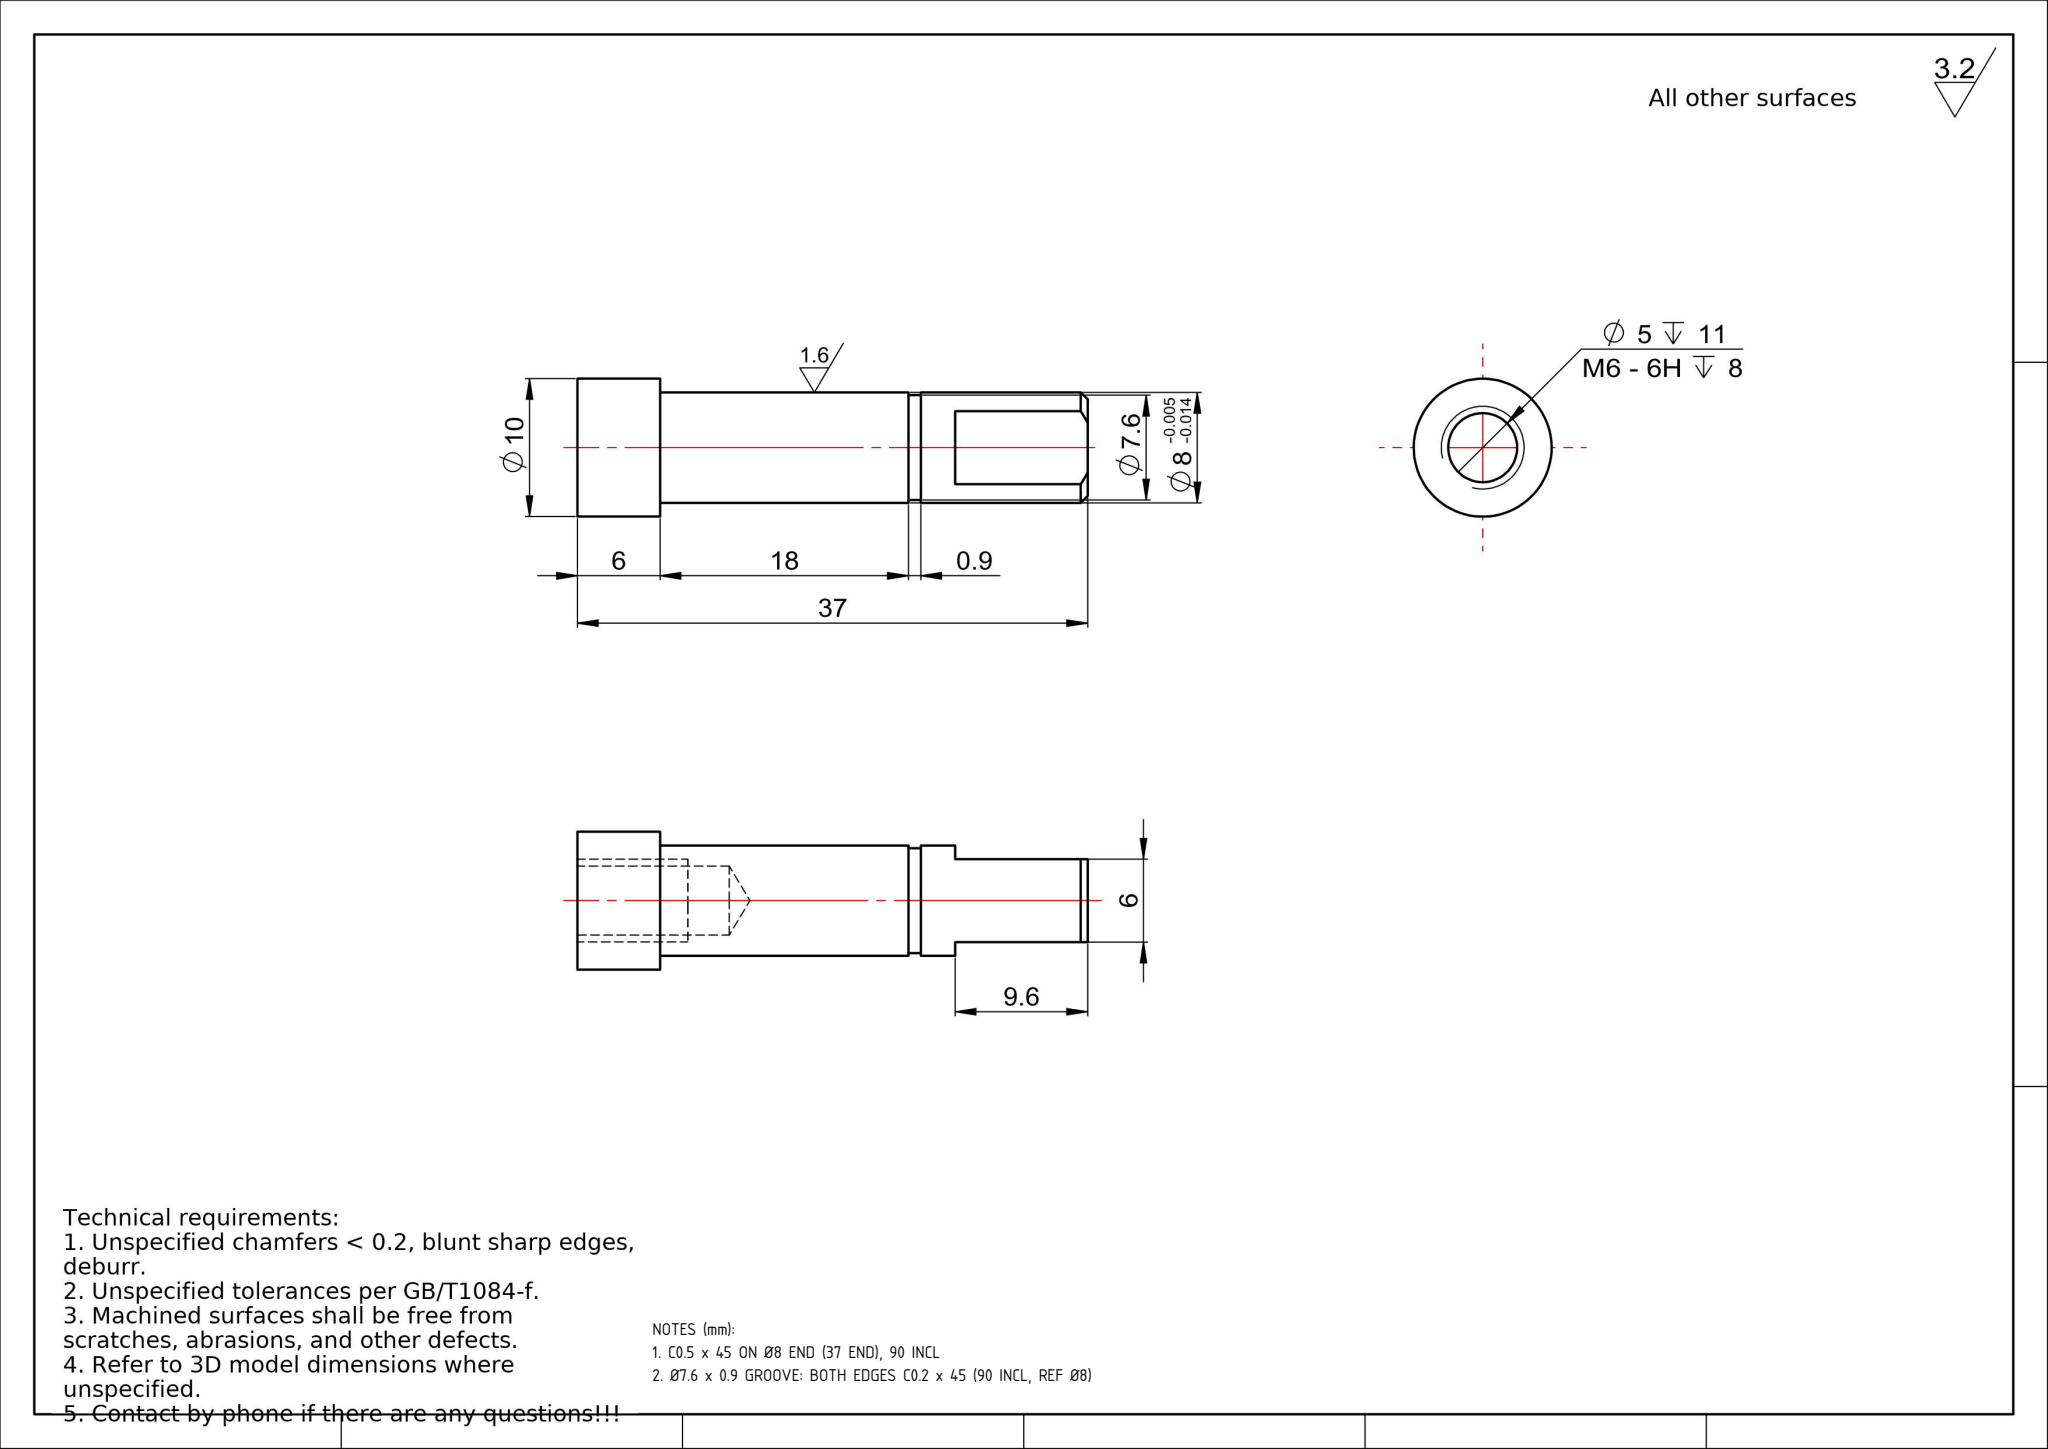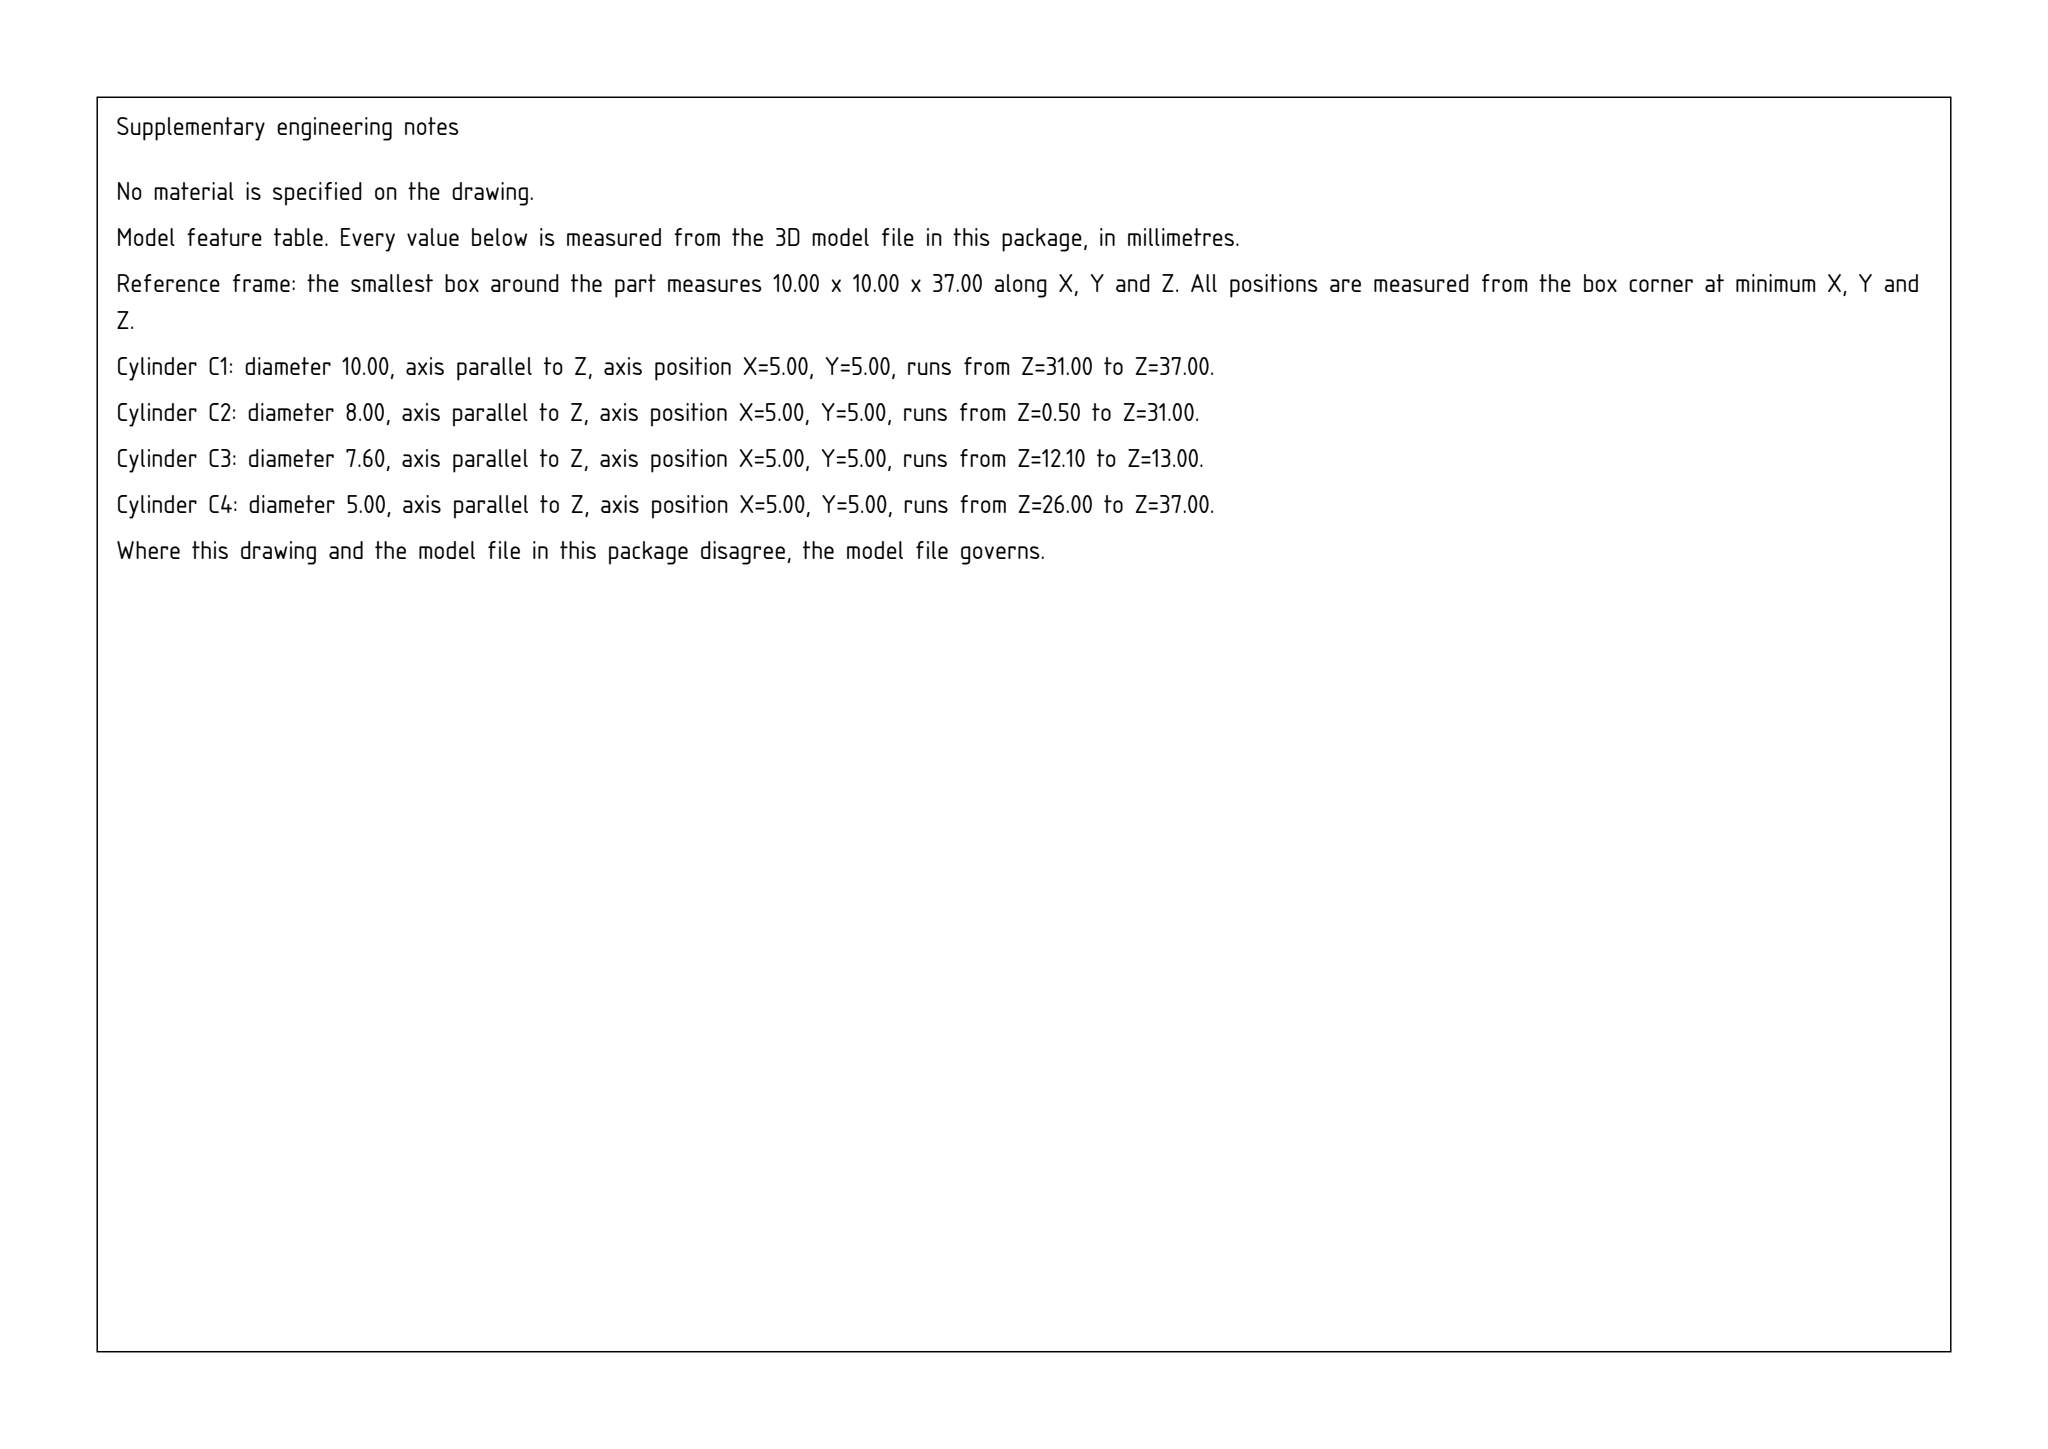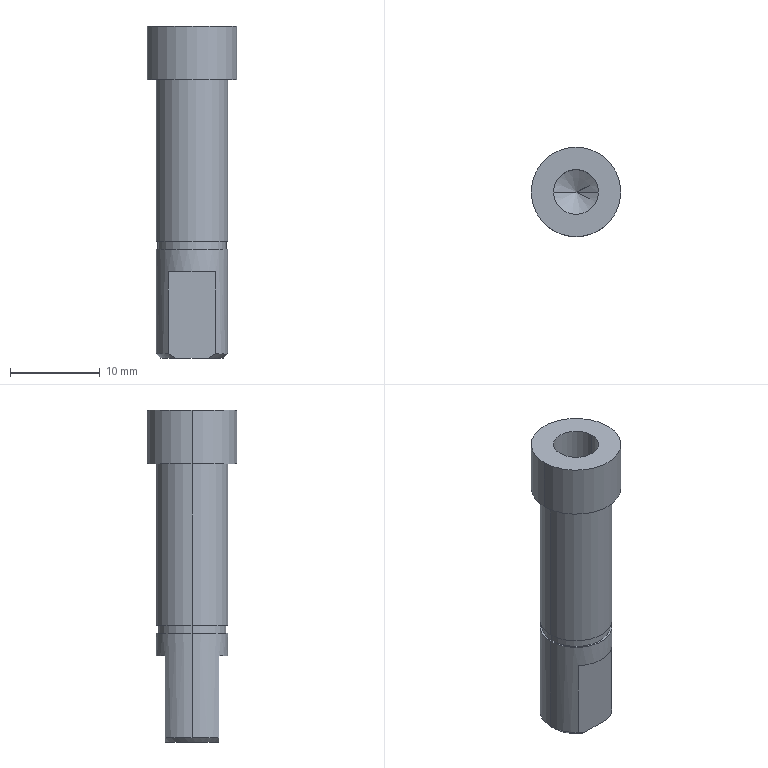Part | SolidWorks | mm | 1 solid | 24 faces | box 10 x 10 x 37 mm | volume 1728 mm3 | cylinder 10 | plane 9 | cone 5 | commonest cylinder face diameters 8 x4 5 x2 10 x2 7.6 x2
Drawing notes:
C0.5 x 45 ON Ø8 END (37 END), 90 INCL | from the solid: cones[included_angle,ref_dia]=90.0 @ ref dia 8.0 at z=37 end face of Ø8 shaft
Ø7.6 x 0.9 GROOVE: BOTH EDGES C0.2 x 45 (90 INCL, REF Ø8) | from the solid: cyl Ø7.6 L0.9 between z=12.1 and 13.0; 90 deg cones ref Ø8; (8-7.6)/2=0.2 radial
build123d program:
from build123d import *

# Parameters (mm, degrees)
SKETCH1_R               = 4
BOSS_EXTRUDE1_DEPTH     = 12.1
SKETCH2_R               = 3.8
BOSS_EXTRUDE2_DEPTH     = 0.9
SKETCH3_R               = 4
BOSS_EXTRUDE3_DEPTH     = 18
SKETCH4_R               = 5
BOSS_EXTRUDE4_DEPTH     = 6
M6_TAPPED_HOLE1_D       = 5
M6_TAPPED_HOLE1_DEPTH   = 11
M6_TAPPED_HOLE1_TIP     = 1.502
CHAMFER3_SIZE           = 0.5
CUT_EXTRUDE3_DEPTH      = 8.5
CUT_EXTRUDE3_DEPTH_BACK = 10.5
SKETCH12_W              = 11.607
SKETCH12_H              = 3.001


with BuildPart() as part:
    # Sketch1 → Boss-Extrude1 (new body)
    with BuildSketch(Plane.XY):
        Circle(SKETCH1_R)
    extrude(amount=BOSS_EXTRUDE1_DEPTH)

    # Sketch2 → Boss-Extrude2 (add)
    with BuildSketch(Plane.XY.offset(12.1)):
        Circle(SKETCH2_R)
    extrude(amount=BOSS_EXTRUDE2_DEPTH)

    # Sketch3 → Boss-Extrude3 (add)
    with BuildSketch(Plane.XY.offset(13)):
        Circle(SKETCH3_R)
    extrude(amount=BOSS_EXTRUDE3_DEPTH)

    # Sketch4 → Boss-Extrude4 (add)
    with BuildSketch(Plane.XY.offset(31)):
        Circle(SKETCH4_R)
    extrude(amount=BOSS_EXTRUDE4_DEPTH)

    # M6 Tapped Hole1
    with Locations(Plane.XY.offset(37)):
        with Locations((0, 0)):
            Hole(M6_TAPPED_HOLE1_D / 2, depth=M6_TAPPED_HOLE1_DEPTH)
            with Locations((0, 0, -(M6_TAPPED_HOLE1_DEPTH + M6_TAPPED_HOLE1_TIP / 2))):  # 118° drill point
                Cone(0, M6_TAPPED_HOLE1_D / 2, M6_TAPPED_HOLE1_TIP, mode=Mode.SUBTRACT)

    # Chamfer3
    chamfer3_edges = [part.edges().sort_by_distance(p)[0] for p in [
        (-4, 0, 0),
    ]]
    chamfer(chamfer3_edges, length=CHAMFER3_SIZE)

    # Sketch12 → Cut-Extrude3 (cut, two sides: drawn at the far end of the back side and taken through both)
    with BuildSketch(Plane(origin=(0, 0, 0), x_dir=(0, 0, -1), z_dir=(1, 0, 0)).offset(-CUT_EXTRUDE3_DEPTH_BACK)):
        with Locations((-3.796, 4.5)):
            Rectangle(SKETCH12_W, SKETCH12_H)
        with Locations((-3.796, -4.5)):
            Rectangle(SKETCH12_W, SKETCH12_H)
    extrude(amount=CUT_EXTRUDE3_DEPTH + CUT_EXTRUDE3_DEPTH_BACK, mode=Mode.SUBTRACT)


solid = part.part
STEP:
#1=CARTESIAN_POINT('',(3.5,0.,0.));
#2=VERTEX_POINT('',#1);
#3=CARTESIAN_POINT('',(1.803,-3.,0.));
#4=VERTEX_POINT('',#3);
#5=CARTESIAN_POINT('',(0.,0.,0.));
#6=DIRECTION('',(0.,0.,-1.));
#7=DIRECTION('',(1.,0.,0.));
#8=AXIS2_PLACEMENT_3D('',#5,#6,#7);
#9=CIRCLE('',#8,3.5);
#10=EDGE_CURVE('',#2,#4,#9,.T.);
#11=ORIENTED_EDGE('',*,*,#10,.F.);
#12=CARTESIAN_POINT('',(4.,0.,0.5));
#13=VERTEX_POINT('',#12);
#14=CARTESIAN_POINT('',(4.,0.,0.5));
#15=DIRECTION('',(0.7071,0.,0.7071));
#16=VECTOR('',#15,1000.);
#17=LINE('',#14,#16);
#18=EDGE_CURVE('',#2,#13,#17,.T.);
#19=ORIENTED_EDGE('',*,*,#18,.T.);
#20=CARTESIAN_POINT('',(2.646,-3.,0.5));
#21=VERTEX_POINT('',#20);
#22=CARTESIAN_POINT('',(0.,0.,0.5));
#23=DIRECTION('',(0.,0.,1.));
#24=DIRECTION('',(1.,0.,0.));
#25=AXIS2_PLACEMENT_3D('',#22,#23,#24);
#26=CIRCLE('',#25,4.);
#27=EDGE_CURVE('',#21,#13,#26,.T.);
#28=ORIENTED_EDGE('',*,*,#27,.F.);
#29=CARTESIAN_POINT('',(1.803,-3.,0.));
#30=CARTESIAN_POINT('',(2.092,-3.,0.1492));
#31=CARTESIAN_POINT('',(2.373,-3.,0.3199));
#32=CARTESIAN_POINT('',(2.646,-3.,0.5));
#33=B_SPLINE_CURVE_WITH_KNOTS('',3,(#29,#30,#31,#32),.UNSPECIFIED.,.F.,.F.,(4,4),(0.01215,0.01313),.UNSPECIFIED.);
#34=EDGE_CURVE('',#4,#21,#33,.T.);
#35=ORIENTED_EDGE('',*,*,#34,.F.);
#36=EDGE_LOOP('',(#11,#19,#28,#35));
#37=FACE_OUTER_BOUND('',#36,.T.);
#38=CARTESIAN_POINT('',(0.,0.,0.5));
#39=DIRECTION('',(0.,0.,1.));
#40=DIRECTION('',(1.,0.,0.));
#41=AXIS2_PLACEMENT_3D('',#38,#39,#40);
#42=CONICAL_SURFACE('',#41,4.,0.7854);
#43=ADVANCED_FACE('',(#37),#42,.T.);
#44=CARTESIAN_POINT('',(-2.5,0.,26.));
#45=VERTEX_POINT('',#44);
#46=CARTESIAN_POINT('',(2.5,0.,26.));
#47=VERTEX_POINT('',#46);
#48=CARTESIAN_POINT('',(0.,0.,26.));
#49=DIRECTION('',(0.,0.,1.));
#50=DIRECTION('',(1.,0.,0.));
#51=AXIS2_PLACEMENT_3D('',#48,#49,#50);
#52=CIRCLE('',#51,2.5);
#53=EDGE_CURVE('',#45,#47,#52,.T.);
#54=ORIENTED_EDGE('',*,*,#53,.F.);
#55=CARTESIAN_POINT('',(-2.5,0.,37.));
#56=VERTEX_POINT('',#55);
#57=CARTESIAN_POINT('',(-2.5,0.,37.));
#58=DIRECTION('',(0.,0.,1.));
#59=VECTOR('',#58,1000.);
#60=LINE('',#57,#59);
#61=EDGE_CURVE('',#45,#56,#60,.T.);
#62=ORIENTED_EDGE('',*,*,#61,.T.);
#63=CARTESIAN_POINT('',(2.5,0.,37.));
#64=VERTEX_POINT('',#63);
#65=CARTESIAN_POINT('',(0.,0.,37.));
#66=DIRECTION('',(0.,0.,1.));
#67=DIRECTION('',(1.,0.,0.));
#68=AXIS2_PLACEMENT_3D('',#65,#66,#67);
#69=CIRCLE('',#68,2.5);
#70=EDGE_CURVE('',#56,#64,#69,.T.);
#71=ORIENTED_EDGE('',*,*,#70,.T.);
#72=CARTESIAN_POINT('',(2.5,0.,37.));
#73=DIRECTION('',(0.,0.,1.));
#74=VECTOR('',#73,1000.);
#75=LINE('',#72,#74);
#76=EDGE_CURVE('',#47,#64,#75,.T.);
#77=ORIENTED_EDGE('',*,*,#76,.F.);
#78=EDGE_LOOP('',(#54,#62,#71,#77));
#79=FACE_OUTER_BOUND('',#78,.T.);
#80=CARTESIAN_POINT('',(0.,0.,37.));
#81=DIRECTION('',(0.,0.,1.));
#82=DIRECTION('',(1.,0.,0.));
#83=AXIS2_PLACEMENT_3D('',#80,#81,#82);
#84=CYLINDRICAL_SURFACE('',#83,2.5);
#85=ADVANCED_FACE('',(#79),#84,.F.);
#86=CARTESIAN_POINT('',(-0.,0.,24.498));
#87=VERTEX_POINT('',#86);
#88=CARTESIAN_POINT('',(2.5,0.,26.));
#89=DIRECTION('',(0.8572,0.,0.515));
#90=VECTOR('',#89,1000.);
#91=LINE('',#88,#90);
#92=EDGE_CURVE('',#87,#47,#91,.T.);
#93=ORIENTED_EDGE('',*,*,#92,.F.);
#94=CARTESIAN_POINT('',(-2.5,0.,26.));
#95=DIRECTION('',(-0.8572,0.,0.515));
#96=VECTOR('',#95,1000.);
#97=LINE('',#94,#96);
#98=EDGE_CURVE('',#87,#45,#97,.T.);
#99=ORIENTED_EDGE('',*,*,#98,.T.);
#100=ORIENTED_EDGE('',*,*,#53,.T.);
#101=EDGE_LOOP('',(#93,#99,#100));
#102=FACE_OUTER_BOUND('',#101,.T.);
#103=CARTESIAN_POINT('',(0.,0.,26.));
#104=DIRECTION('',(0.,0.,1.));
#105=DIRECTION('',(1.,0.,0.));
#106=AXIS2_PLACEMENT_3D('',#103,#104,#105);
#107=CONICAL_SURFACE('',#106,2.5,1.03);
#108=ADVANCED_FACE('',(#102),#107,.F.);
#109=CARTESIAN_POINT('',(5.,0.,37.));
#110=VERTEX_POINT('',#109);
#111=CARTESIAN_POINT('',(-5.,0.,37.));
#112=VERTEX_POINT('',#111);
#113=CARTESIAN_POINT('',(0.,0.,37.));
#114=DIRECTION('',(0.,0.,1.));
#115=DIRECTION('',(1.,0.,0.));
#116=AXIS2_PLACEMENT_3D('',#113,#114,#115);
#117=CIRCLE('',#116,5.);
#118=EDGE_CURVE('',#110,#112,#117,.T.);
#119=ORIENTED_EDGE('',*,*,#118,.F.);
#120=CARTESIAN_POINT('',(5.,0.,31.));
#121=VERTEX_POINT('',#120);
#122=CARTESIAN_POINT('',(5.,0.,37.));
#123=DIRECTION('',(0.,0.,-1.));
#124=VECTOR('',#123,1000.);
#125=LINE('',#122,#124);
#126=EDGE_CURVE('',#110,#121,#125,.T.);
#127=ORIENTED_EDGE('',*,*,#126,.T.);
#128=CARTESIAN_POINT('',(-5.,0.,31.));
#129=VERTEX_POINT('',#128);
#130=CARTESIAN_POINT('',(0.,0.,31.));
#131=DIRECTION('',(0.,0.,1.));
#132=DIRECTION('',(1.,0.,0.));
#133=AXIS2_PLACEMENT_3D('',#130,#131,#132);
#134=CIRCLE('',#133,5.);
#135=EDGE_CURVE('',#121,#129,#134,.T.);
#136=ORIENTED_EDGE('',*,*,#135,.T.);
#137=CARTESIAN_POINT('',(-5.,0.,37.));
#138=DIRECTION('',(0.,0.,-1.));
#139=VECTOR('',#138,1000.);
#140=LINE('',#137,#139);
#141=EDGE_CURVE('',#112,#129,#140,.T.);
#142=ORIENTED_EDGE('',*,*,#141,.F.);
#143=EDGE_LOOP('',(#119,#127,#136,#142));
#144=FACE_OUTER_BOUND('',#143,.T.);
#145=CARTESIAN_POINT('',(0.,0.,37.));
#146=DIRECTION('',(0.,0.,-1.));
#147=DIRECTION('',(-1.,0.,0.));
#148=AXIS2_PLACEMENT_3D('',#145,#146,#147);
#149=CYLINDRICAL_SURFACE('',#148,5.);
#150=ADVANCED_FACE('',(#144),#149,.T.);
#151=CARTESIAN_POINT('',(4.,0.,31.));
#152=VERTEX_POINT('',#151);
#153=CARTESIAN_POINT('',(-4.,0.,31.));
#154=VERTEX_POINT('',#153);
#155=CARTESIAN_POINT('',(0.,0.,31.));
#156=DIRECTION('',(0.,0.,1.));
#157=DIRECTION('',(1.,0.,0.));
#158=AXIS2_PLACEMENT_3D('',#155,#156,#157);
#159=CIRCLE('',#158,4.);
#160=EDGE_CURVE('',#152,#154,#159,.T.);
#161=ORIENTED_EDGE('',*,*,#160,.F.);
#162=CARTESIAN_POINT('',(4.,0.,13.));
#163=VERTEX_POINT('',#162);
#164=CARTESIAN_POINT('',(4.,0.,31.));
#165=DIRECTION('',(0.,0.,-1.));
#166=VECTOR('',#165,1000.);
#167=LINE('',#164,#166);
#168=EDGE_CURVE('',#152,#163,#167,.T.);
#169=ORIENTED_EDGE('',*,*,#168,.T.);
#170=CARTESIAN_POINT('',(-4.,0.,13.));
#171=VERTEX_POINT('',#170);
#172=CARTESIAN_POINT('',(0.,0.,13.));
#173=DIRECTION('',(0.,0.,1.));
#174=DIRECTION('',(1.,0.,0.));
#175=AXIS2_PLACEMENT_3D('',#172,#173,#174);
#176=CIRCLE('',#175,4.);
#177=EDGE_CURVE('',#163,#171,#176,.T.);
#178=ORIENTED_EDGE('',*,*,#177,.T.);
#179=CARTESIAN_POINT('',(-4.,0.,31.));
#180=DIRECTION('',(0.,0.,-1.));
#181=VECTOR('',#180,1000.);
#182=LINE('',#179,#181);
#183=EDGE_CURVE('',#154,#171,#182,.T.);
#184=ORIENTED_EDGE('',*,*,#183,.F.);
#185=EDGE_LOOP('',(#161,#169,#178,#184));
#186=FACE_OUTER_BOUND('',#185,.T.);
#187=CARTESIAN_POINT('',(0.,0.,31.));
#188=DIRECTION('',(0.,0.,-1.));
#189=DIRECTION('',(-1.,0.,0.));
#190=AXIS2_PLACEMENT_3D('',#187,#188,#189);
#191=CYLINDRICAL_SURFACE('',#190,4.);
#192=ADVANCED_FACE('',(#186),#191,.T.);
#193=CARTESIAN_POINT('',(3.8,0.,13.));
#194=VERTEX_POINT('',#193);
#195=CARTESIAN_POINT('',(-3.8,0.,13.));
#196=VERTEX_POINT('',#195);
#197=CARTESIAN_POINT('',(0.,0.,13.));
#198=DIRECTION('',(0.,0.,1.));
#199=DIRECTION('',(1.,0.,0.));
#200=AXIS2_PLACEMENT_3D('',#197,#198,#199);
#201=CIRCLE('',#200,3.8);
#202=EDGE_CURVE('',#194,#196,#201,.T.);
#203=ORIENTED_EDGE('',*,*,#202,.F.);
#204=CARTESIAN_POINT('',(3.8,0.,12.1));
#205=VERTEX_POINT('',#204);
#206=CARTESIAN_POINT('',(3.8,0.,13.));
#207=DIRECTION('',(0.,0.,-1.));
#208=VECTOR('',#207,1000.);
#209=LINE('',#206,#208);
#210=EDGE_CURVE('',#194,#205,#209,.T.);
#211=ORIENTED_EDGE('',*,*,#210,.T.);
#212=CARTESIAN_POINT('',(-3.8,0.,12.1));
#213=VERTEX_POINT('',#212);
#214=CARTESIAN_POINT('',(0.,0.,12.1));
#215=DIRECTION('',(0.,0.,1.));
#216=DIRECTION('',(1.,0.,0.));
#217=AXIS2_PLACEMENT_3D('',#214,#215,#216);
#218=CIRCLE('',#217,3.8);
#219=EDGE_CURVE('',#205,#213,#218,.T.);
#220=ORIENTED_EDGE('',*,*,#219,.T.);
#221=CARTESIAN_POINT('',(-3.8,0.,13.));
#222=DIRECTION('',(0.,0.,-1.));
#223=VECTOR('',#222,1000.);
#224=LINE('',#221,#223);
#225=EDGE_CURVE('',#196,#213,#224,.T.);
#226=ORIENTED_EDGE('',*,*,#225,.F.);
#227=EDGE_LOOP('',(#203,#211,#220,#226));
#228=FACE_OUTER_BOUND('',#227,.T.);
#229=CARTESIAN_POINT('',(0.,0.,13.));
#230=DIRECTION('',(0.,0.,-1.));
#231=DIRECTION('',(-1.,0.,0.));
#232=AXIS2_PLACEMENT_3D('',#229,#230,#231);
#233=CYLINDRICAL_SURFACE('',#232,3.8);
#234=ADVANCED_FACE('',(#228),#233,.T.);
#235=CARTESIAN_POINT('',(4.,0.,12.1));
#236=VERTEX_POINT('',#235);
#237=CARTESIAN_POINT('',(-4.,0.,12.1));
#238=VERTEX_POINT('',#237);
#239=CARTESIAN_POINT('',(0.,0.,12.1));
#240=DIRECTION('',(0.,0.,1.));
#241=DIRECTION('',(1.,0.,0.));
#242=AXIS2_PLACEMENT_3D('',#239,#240,#241);
#243=CIRCLE('',#242,4.);
#244=EDGE_CURVE('',#236,#238,#243,.T.);
#245=ORIENTED_EDGE('',*,*,#244,.F.);
#246=CARTESIAN_POINT('',(4.,0.,12.1));
#247=DIRECTION('',(0.,0.,-1.));
#248=VECTOR('',#247,1000.);
#249=LINE('',#246,#248);
#250=EDGE_CURVE('',#236,#13,#249,.T.);
#251=ORIENTED_EDGE('',*,*,#250,.T.);
#252=CARTESIAN_POINT('',(2.646,3.,0.5));
#253=VERTEX_POINT('',#252);
#254=CARTESIAN_POINT('',(0.,0.,0.5));
#255=DIRECTION('',(0.,0.,1.));
#256=DIRECTION('',(1.,0.,0.));
#257=AXIS2_PLACEMENT_3D('',#254,#255,#256);
#258=CIRCLE('',#257,4.);
#259=EDGE_CURVE('',#13,#253,#258,.T.);
#260=ORIENTED_EDGE('',*,*,#259,.T.);
#261=CARTESIAN_POINT('',(2.646,3.,9.6));
#262=VERTEX_POINT('',#261);
#263=CARTESIAN_POINT('',(2.646,3.,12.1));
#264=DIRECTION('',(0.,0.,1.));
#265=VECTOR('',#264,1000.);
#266=LINE('',#263,#265);
#267=EDGE_CURVE('',#253,#262,#266,.T.);
#268=ORIENTED_EDGE('',*,*,#267,.T.);
#269=CARTESIAN_POINT('',(-2.646,3.,9.6));
#270=VERTEX_POINT('',#269);
#271=CARTESIAN_POINT('',(0.,0.,9.6));
#272=DIRECTION('',(0.,-0.,1.));
#273=DIRECTION('',(0.,-1.,-0.));
#274=AXIS2_PLACEMENT_3D('',#271,#272,#273);
#275=CIRCLE('',#274,4.);
#276=EDGE_CURVE('',#262,#270,#275,.T.);
#277=ORIENTED_EDGE('',*,*,#276,.T.);
#278=CARTESIAN_POINT('',(-2.646,3.,0.5));
#279=VERTEX_POINT('',#278);
#280=CARTESIAN_POINT('',(-2.646,3.,12.1));
#281=DIRECTION('',(0.,0.,-1.));
#282=VECTOR('',#281,1000.);
#283=LINE('',#280,#282);
#284=EDGE_CURVE('',#270,#279,#283,.T.);
#285=ORIENTED_EDGE('',*,*,#284,.T.);
#286=CARTESIAN_POINT('',(-4.,0.,0.5));
#287=VERTEX_POINT('',#286);
#288=CARTESIAN_POINT('',(0.,0.,0.5));
#289=DIRECTION('',(0.,0.,1.));
#290=DIRECTION('',(1.,0.,0.));
#291=AXIS2_PLACEMENT_3D('',#288,#289,#290);
#292=CIRCLE('',#291,4.);
#293=EDGE_CURVE('',#279,#287,#292,.T.);
#294=ORIENTED_EDGE('',*,*,#293,.T.);
#295=CARTESIAN_POINT('',(-4.,0.,12.1));
#296=DIRECTION('',(0.,0.,-1.));
#297=VECTOR('',#296,1000.);
#298=LINE('',#295,#297);
#299=EDGE_CURVE('',#238,#287,#298,.T.);
#300=ORIENTED_EDGE('',*,*,#299,.F.);
#301=EDGE_LOOP('',(#245,#251,#260,#268,#277,#285,#294,#300));
#302=FACE_OUTER_BOUND('',#301,.T.);
#303=CARTESIAN_POINT('',(0.,0.,12.1));
#304=DIRECTION('',(0.,0.,-1.));
#305=DIRECTION('',(-1.,0.,0.));
#306=AXIS2_PLACEMENT_3D('',#303,#304,#305);
#307=CYLINDRICAL_SURFACE('',#306,4.);
#308=ADVANCED_FACE('',(#302),#307,.T.);
#309=CARTESIAN_POINT('',(-2.646,-3.,0.5));
#310=VERTEX_POINT('',#309);
#311=CARTESIAN_POINT('',(-1.803,-3.,0.));
#312=VERTEX_POINT('',#311);
#313=CARTESIAN_POINT('',(-2.646,-3.,0.5));
#314=CARTESIAN_POINT('',(-2.374,-3.,0.3203));
#315=CARTESIAN_POINT('',(-2.095,-3.,0.1506));
#316=CARTESIAN_POINT('',(-1.803,-3.,0.));
#317=B_SPLINE_CURVE_WITH_KNOTS('',3,(#313,#314,#315,#316),.UNSPECIFIED.,.F.,.F.,(4,4),(0.007424,0.008405),.UNSPECIFIED.);
#318=EDGE_CURVE('',#310,#312,#317,.T.);
#319=ORIENTED_EDGE('',*,*,#318,.F.);
#320=CARTESIAN_POINT('',(0.,0.,0.5));
#321=DIRECTION('',(0.,0.,1.));
#322=DIRECTION('',(1.,0.,0.));
#323=AXIS2_PLACEMENT_3D('',#320,#321,#322);
#324=CIRCLE('',#323,4.);
#325=EDGE_CURVE('',#287,#310,#324,.T.);
#326=ORIENTED_EDGE('',*,*,#325,.F.);
#327=ORIENTED_EDGE('',*,*,#293,.F.);
#328=CARTESIAN_POINT('',(-1.803,3.,0.));
#329=VERTEX_POINT('',#328);
#330=CARTESIAN_POINT('',(-1.803,3.,0.));
#331=CARTESIAN_POINT('',(-2.092,3.,0.1492));
#332=CARTESIAN_POINT('',(-2.373,3.,0.3199));
#333=CARTESIAN_POINT('',(-2.646,3.,0.5));
#334=B_SPLINE_CURVE_WITH_KNOTS('',3,(#330,#331,#332,#333),.UNSPECIFIED.,.F.,.F.,(4,4),(0.01215,0.01313),.UNSPECIFIED.);
#335=EDGE_CURVE('',#329,#279,#334,.T.);
#336=ORIENTED_EDGE('',*,*,#335,.F.);
#337=CARTESIAN_POINT('',(0.,0.,0.));
#338=DIRECTION('',(0.,0.,-1.));
#339=DIRECTION('',(1.,0.,0.));
#340=AXIS2_PLACEMENT_3D('',#337,#338,#339);
#341=CIRCLE('',#340,3.5);
#342=EDGE_CURVE('',#312,#329,#341,.T.);
#343=ORIENTED_EDGE('',*,*,#342,.F.);
#344=EDGE_LOOP('',(#319,#326,#327,#336,#343));
#345=FACE_OUTER_BOUND('',#344,.T.);
#346=CARTESIAN_POINT('',(0.,0.,0.5));
#347=DIRECTION('',(0.,0.,1.));
#348=DIRECTION('',(1.,0.,0.));
#349=AXIS2_PLACEMENT_3D('',#346,#347,#348);
#350=CONICAL_SURFACE('',#349,4.,0.7854);
#351=ADVANCED_FACE('',(#345),#350,.T.);
#352=ORIENTED_EDGE('',*,*,#250,.F.);
#353=CARTESIAN_POINT('',(0.,0.,12.1));
#354=DIRECTION('',(0.,0.,1.));
#355=DIRECTION('',(1.,0.,0.));
#356=AXIS2_PLACEMENT_3D('',#353,#354,#355);
#357=CIRCLE('',#356,4.);
#358=EDGE_CURVE('',#238,#236,#357,.T.);
#359=ORIENTED_EDGE('',*,*,#358,.F.);
#360=ORIENTED_EDGE('',*,*,#299,.T.);
#361=ORIENTED_EDGE('',*,*,#325,.T.);
#362=CARTESIAN_POINT('',(-2.646,-3.,9.6));
#363=VERTEX_POINT('',#362);
#364=CARTESIAN_POINT('',(-2.646,-3.,12.1));
#365=DIRECTION('',(0.,0.,1.));
#366=VECTOR('',#365,1000.);
#367=LINE('',#364,#366);
#368=EDGE_CURVE('',#310,#363,#367,.T.);
#369=ORIENTED_EDGE('',*,*,#368,.T.);
#370=CARTESIAN_POINT('',(2.646,-3.,9.6));
#371=VERTEX_POINT('',#370);
#372=CARTESIAN_POINT('',(0.,0.,9.6));
#373=DIRECTION('',(0.,0.,1.));
#374=DIRECTION('',(0.,-1.,0.));
#375=AXIS2_PLACEMENT_3D('',#372,#373,#374);
#376=CIRCLE('',#375,4.);
#377=EDGE_CURVE('',#363,#371,#376,.T.);
#378=ORIENTED_EDGE('',*,*,#377,.T.);
#379=CARTESIAN_POINT('',(2.646,-3.,12.1));
#380=DIRECTION('',(0.,0.,-1.));
#381=VECTOR('',#380,1000.);
#382=LINE('',#379,#381);
#383=EDGE_CURVE('',#371,#21,#382,.T.);
#384=ORIENTED_EDGE('',*,*,#383,.T.);
#385=ORIENTED_EDGE('',*,*,#27,.T.);
#386=EDGE_LOOP('',(#352,#359,#360,#361,#369,#378,#384,#385));
#387=FACE_OUTER_BOUND('',#386,.T.);
#388=CARTESIAN_POINT('',(0.,0.,12.1));
#389=DIRECTION('',(0.,0.,-1.));
#390=DIRECTION('',(-1.,0.,0.));
#391=AXIS2_PLACEMENT_3D('',#388,#389,#390);
#392=CYLINDRICAL_SURFACE('',#391,4.);
#393=ADVANCED_FACE('',(#387),#392,.T.);
#394=CARTESIAN_POINT('',(0.,0.,12.1));
#395=DIRECTION('',(0.,0.,1.));
#396=DIRECTION('',(1.,0.,0.));
#397=AXIS2_PLACEMENT_3D('',#394,#395,#396);
#398=CIRCLE('',#397,3.8);
#399=EDGE_CURVE('',#213,#205,#398,.T.);
#400=ORIENTED_EDGE('',*,*,#399,.F.);
#401=ORIENTED_EDGE('',*,*,#219,.F.);
#402=EDGE_LOOP('',(#400,#401));
#403=FACE_BOUND('',#402,.T.);
#404=ORIENTED_EDGE('',*,*,#358,.T.);
#405=ORIENTED_EDGE('',*,*,#244,.T.);
#406=EDGE_LOOP('',(#404,#405));
#407=FACE_OUTER_BOUND('',#406,.T.);
#408=CARTESIAN_POINT('',(0.,0.,12.1));
#409=DIRECTION('',(0.,0.,1.));
#410=DIRECTION('',(1.,0.,0.));
#411=AXIS2_PLACEMENT_3D('',#408,#409,#410);
#412=PLANE('',#411);
#413=ADVANCED_FACE('',(#403,#407),#412,.T.);
#414=CARTESIAN_POINT('',(1.803,3.,0.));
#415=VERTEX_POINT('',#414);
#416=CARTESIAN_POINT('',(0.,0.,0.));
#417=DIRECTION('',(0.,0.,-1.));
#418=DIRECTION('',(1.,0.,0.));
#419=AXIS2_PLACEMENT_3D('',#416,#417,#418);
#420=CIRCLE('',#419,3.5);
#421=EDGE_CURVE('',#415,#2,#420,.T.);
#422=ORIENTED_EDGE('',*,*,#421,.T.);
#423=ORIENTED_EDGE('',*,*,#10,.T.);
#424=CARTESIAN_POINT('',(0.,-3.,0.));
#425=DIRECTION('',(-1.,0.,0.));
#426=VECTOR('',#425,1000.);
#427=LINE('',#424,#426);
#428=EDGE_CURVE('',#4,#312,#427,.T.);
#429=ORIENTED_EDGE('',*,*,#428,.T.);
#430=ORIENTED_EDGE('',*,*,#342,.T.);
#431=CARTESIAN_POINT('',(0.,3.,0.));
#432=DIRECTION('',(1.,0.,0.));
#433=VECTOR('',#432,1000.);
#434=LINE('',#431,#433);
#435=EDGE_CURVE('',#329,#415,#434,.T.);
#436=ORIENTED_EDGE('',*,*,#435,.T.);
#437=EDGE_LOOP('',(#422,#423,#429,#430,#436));
#438=FACE_OUTER_BOUND('',#437,.T.);
#439=CARTESIAN_POINT('',(0.,0.,0.));
#440=DIRECTION('',(0.,0.,1.));
#441=DIRECTION('',(1.,0.,0.));
#442=AXIS2_PLACEMENT_3D('',#439,#440,#441);
#443=PLANE('',#442);
#444=ADVANCED_FACE('',(#438),#443,.F.);
#445=ORIENTED_EDGE('',*,*,#210,.F.);
#446=CARTESIAN_POINT('',(0.,0.,13.));
#447=DIRECTION('',(0.,0.,1.));
#448=DIRECTION('',(1.,0.,0.));
#449=AXIS2_PLACEMENT_3D('',#446,#447,#448);
#450=CIRCLE('',#449,3.8);
#451=EDGE_CURVE('',#196,#194,#450,.T.);
#452=ORIENTED_EDGE('',*,*,#451,.F.);
#453=ORIENTED_EDGE('',*,*,#225,.T.);
#454=ORIENTED_EDGE('',*,*,#399,.T.);
#455=EDGE_LOOP('',(#445,#452,#453,#454));
#456=FACE_OUTER_BOUND('',#455,.T.);
#457=CARTESIAN_POINT('',(0.,0.,13.));
#458=DIRECTION('',(0.,0.,-1.));
#459=DIRECTION('',(-1.,0.,0.));
#460=AXIS2_PLACEMENT_3D('',#457,#458,#459);
#461=CYLINDRICAL_SURFACE('',#460,3.8);
#462=ADVANCED_FACE('',(#456),#461,.T.);
#463=ORIENTED_EDGE('',*,*,#168,.F.);
#464=CARTESIAN_POINT('',(0.,0.,31.));
#465=DIRECTION('',(0.,0.,1.));
#466=DIRECTION('',(1.,0.,0.));
#467=AXIS2_PLACEMENT_3D('',#464,#465,#466);
#468=CIRCLE('',#467,4.);
#469=EDGE_CURVE('',#154,#152,#468,.T.);
#470=ORIENTED_EDGE('',*,*,#469,.F.);
#471=ORIENTED_EDGE('',*,*,#183,.T.);
#472=CARTESIAN_POINT('',(0.,0.,13.));
#473=DIRECTION('',(0.,0.,1.));
#474=DIRECTION('',(1.,0.,0.));
#475=AXIS2_PLACEMENT_3D('',#472,#473,#474);
#476=CIRCLE('',#475,4.);
#477=EDGE_CURVE('',#171,#163,#476,.T.);
#478=ORIENTED_EDGE('',*,*,#477,.T.);
#479=EDGE_LOOP('',(#463,#470,#471,#478));
#480=FACE_OUTER_BOUND('',#479,.T.);
#481=CARTESIAN_POINT('',(0.,0.,31.));
#482=DIRECTION('',(0.,0.,-1.));
#483=DIRECTION('',(-1.,0.,0.));
#484=AXIS2_PLACEMENT_3D('',#481,#482,#483);
#485=CYLINDRICAL_SURFACE('',#484,4.);
#486=ADVANCED_FACE('',(#480),#485,.T.);
#487=ORIENTED_EDGE('',*,*,#451,.T.);
#488=ORIENTED_EDGE('',*,*,#202,.T.);
#489=EDGE_LOOP('',(#487,#488));
#490=FACE_BOUND('',#489,.T.);
#491=ORIENTED_EDGE('',*,*,#477,.F.);
#492=ORIENTED_EDGE('',*,*,#177,.F.);
#493=EDGE_LOOP('',(#491,#492));
#494=FACE_OUTER_BOUND('',#493,.T.);
#495=CARTESIAN_POINT('',(0.,0.,13.));
#496=DIRECTION('',(0.,0.,1.));
#497=DIRECTION('',(1.,0.,0.));
#498=AXIS2_PLACEMENT_3D('',#495,#496,#497);
#499=PLANE('',#498);
#500=ADVANCED_FACE('',(#490,#494),#499,.F.);
#501=ORIENTED_EDGE('',*,*,#126,.F.);
#502=CARTESIAN_POINT('',(0.,0.,37.));
#503=DIRECTION('',(0.,0.,1.));
#504=DIRECTION('',(1.,0.,0.));
#505=AXIS2_PLACEMENT_3D('',#502,#503,#504);
#506=CIRCLE('',#505,5.);
#507=EDGE_CURVE('',#112,#110,#506,.T.);
#508=ORIENTED_EDGE('',*,*,#507,.F.);
#509=ORIENTED_EDGE('',*,*,#141,.T.);
#510=CARTESIAN_POINT('',(0.,0.,31.));
#511=DIRECTION('',(0.,0.,1.));
#512=DIRECTION('',(1.,0.,0.));
#513=AXIS2_PLACEMENT_3D('',#510,#511,#512);
#514=CIRCLE('',#513,5.);
#515=EDGE_CURVE('',#129,#121,#514,.T.);
#516=ORIENTED_EDGE('',*,*,#515,.T.);
#517=EDGE_LOOP('',(#501,#508,#509,#516));
#518=FACE_OUTER_BOUND('',#517,.T.);
#519=CARTESIAN_POINT('',(0.,0.,37.));
#520=DIRECTION('',(0.,0.,-1.));
#521=DIRECTION('',(-1.,0.,0.));
#522=AXIS2_PLACEMENT_3D('',#519,#520,#521);
#523=CYLINDRICAL_SURFACE('',#522,5.);
#524=ADVANCED_FACE('',(#518),#523,.T.);
#525=CARTESIAN_POINT('',(0.,0.,37.));
#526=DIRECTION('',(0.,0.,1.));
#527=DIRECTION('',(1.,0.,0.));
#528=AXIS2_PLACEMENT_3D('',#525,#526,#527);
#529=CIRCLE('',#528,2.5);
#530=EDGE_CURVE('',#64,#56,#529,.T.);
#531=ORIENTED_EDGE('',*,*,#530,.F.);
#532=ORIENTED_EDGE('',*,*,#70,.F.);
#533=EDGE_LOOP('',(#531,#532));
#534=FACE_BOUND('',#533,.T.);
#535=ORIENTED_EDGE('',*,*,#507,.T.);
#536=ORIENTED_EDGE('',*,*,#118,.T.);
#537=EDGE_LOOP('',(#535,#536));
#538=FACE_OUTER_BOUND('',#537,.T.);
#539=CARTESIAN_POINT('',(0.,0.,37.));
#540=DIRECTION('',(0.,0.,1.));
#541=DIRECTION('',(1.,0.,0.));
#542=AXIS2_PLACEMENT_3D('',#539,#540,#541);
#543=PLANE('',#542);
#544=ADVANCED_FACE('',(#534,#538),#543,.T.);
#545=ORIENTED_EDGE('',*,*,#469,.T.);
#546=ORIENTED_EDGE('',*,*,#160,.T.);
#547=EDGE_LOOP('',(#545,#546));
#548=FACE_BOUND('',#547,.T.);
#549=ORIENTED_EDGE('',*,*,#515,.F.);
#550=ORIENTED_EDGE('',*,*,#135,.F.);
#551=EDGE_LOOP('',(#549,#550));
#552=FACE_OUTER_BOUND('',#551,.T.);
#553=CARTESIAN_POINT('',(0.,0.,31.));
#554=DIRECTION('',(0.,0.,1.));
#555=DIRECTION('',(1.,0.,0.));
#556=AXIS2_PLACEMENT_3D('',#553,#554,#555);
#557=PLANE('',#556);
#558=ADVANCED_FACE('',(#548,#552),#557,.F.);
#559=ORIENTED_EDGE('',*,*,#98,.F.);
#560=ORIENTED_EDGE('',*,*,#92,.T.);
#561=CARTESIAN_POINT('',(0.,0.,26.));
#562=DIRECTION('',(0.,0.,1.));
#563=DIRECTION('',(1.,0.,0.));
#564=AXIS2_PLACEMENT_3D('',#561,#562,#563);
#565=CIRCLE('',#564,2.5);
#566=EDGE_CURVE('',#47,#45,#565,.T.);
#567=ORIENTED_EDGE('',*,*,#566,.T.);
#568=EDGE_LOOP('',(#559,#560,#567));
#569=FACE_OUTER_BOUND('',#568,.T.);
#570=CARTESIAN_POINT('',(0.,0.,26.));
#571=DIRECTION('',(0.,0.,1.));
#572=DIRECTION('',(1.,0.,0.));
#573=AXIS2_PLACEMENT_3D('',#570,#571,#572);
#574=CONICAL_SURFACE('',#573,2.5,1.03);
#575=ADVANCED_FACE('',(#569),#574,.F.);
#576=ORIENTED_EDGE('',*,*,#61,.F.);
#577=ORIENTED_EDGE('',*,*,#566,.F.);
#578=ORIENTED_EDGE('',*,*,#76,.T.);
#579=ORIENTED_EDGE('',*,*,#530,.T.);
#580=EDGE_LOOP('',(#576,#577,#578,#579));
#581=FACE_OUTER_BOUND('',#580,.T.);
#582=CARTESIAN_POINT('',(0.,0.,37.));
#583=DIRECTION('',(0.,0.,1.));
#584=DIRECTION('',(1.,0.,0.));
#585=AXIS2_PLACEMENT_3D('',#582,#583,#584);
#586=CYLINDRICAL_SURFACE('',#585,2.5);
#587=ADVANCED_FACE('',(#581),#586,.F.);
#588=ORIENTED_EDGE('',*,*,#18,.F.);
#589=ORIENTED_EDGE('',*,*,#421,.F.);
#590=CARTESIAN_POINT('',(2.646,3.,0.5));
#591=CARTESIAN_POINT('',(2.374,3.,0.3203));
#592=CARTESIAN_POINT('',(2.095,3.,0.1506));
#593=CARTESIAN_POINT('',(1.803,3.,0.));
#594=B_SPLINE_CURVE_WITH_KNOTS('',3,(#590,#591,#592,#593),.UNSPECIFIED.,.F.,.F.,(4,4),(0.007424,0.008405),.UNSPECIFIED.);
#595=EDGE_CURVE('',#253,#415,#594,.T.);
#596=ORIENTED_EDGE('',*,*,#595,.F.);
#597=ORIENTED_EDGE('',*,*,#259,.F.);
#598=EDGE_LOOP('',(#588,#589,#596,#597));
#599=FACE_OUTER_BOUND('',#598,.T.);
#600=CARTESIAN_POINT('',(0.,0.,0.5));
#601=DIRECTION('',(0.,0.,1.));
#602=DIRECTION('',(1.,0.,0.));
#603=AXIS2_PLACEMENT_3D('',#600,#601,#602);
#604=CONICAL_SURFACE('',#603,4.,0.7854);
#605=ADVANCED_FACE('',(#599),#604,.T.);
#606=CARTESIAN_POINT('',(-10.5,3.,9.6));
#607=DIRECTION('',(1.,0.,0.));
#608=VECTOR('',#607,1000.);
#609=LINE('',#606,#608);
#610=EDGE_CURVE('',#270,#262,#609,.T.);
#611=ORIENTED_EDGE('',*,*,#610,.F.);
#612=ORIENTED_EDGE('',*,*,#276,.F.);
#613=EDGE_LOOP('',(#611,#612));
#614=FACE_OUTER_BOUND('',#613,.T.);
#615=CARTESIAN_POINT('',(-10.5,6.001,9.6));
#616=DIRECTION('',(0.,-0.,1.));
#617=DIRECTION('',(0.,-1.,-0.));
#618=AXIS2_PLACEMENT_3D('',#615,#616,#617);
#619=PLANE('',#618);
#620=ADVANCED_FACE('',(#614),#619,.F.);
#621=ORIENTED_EDGE('',*,*,#595,.T.);
#622=ORIENTED_EDGE('',*,*,#435,.F.);
#623=ORIENTED_EDGE('',*,*,#335,.T.);
#624=ORIENTED_EDGE('',*,*,#284,.F.);
#625=ORIENTED_EDGE('',*,*,#610,.T.);
#626=ORIENTED_EDGE('',*,*,#267,.F.);
#627=EDGE_LOOP('',(#621,#622,#623,#624,#625,#626));
#628=FACE_OUTER_BOUND('',#627,.T.);
#629=CARTESIAN_POINT('',(-10.5,3.,-2.007));
#630=DIRECTION('',(0.,-1.,-0.));
#631=DIRECTION('',(0.,0.,-1.));
#632=AXIS2_PLACEMENT_3D('',#629,#630,#631);
#633=PLANE('',#632);
#634=ADVANCED_FACE('',(#628),#633,.F.);
#635=CARTESIAN_POINT('',(-10.5,-3.,9.6));
#636=DIRECTION('',(1.,0.,0.));
#637=VECTOR('',#636,1000.);
#638=LINE('',#635,#637);
#639=EDGE_CURVE('',#363,#371,#638,.T.);
#640=ORIENTED_EDGE('',*,*,#639,.T.);
#641=ORIENTED_EDGE('',*,*,#377,.F.);
#642=EDGE_LOOP('',(#640,#641));
#643=FACE_OUTER_BOUND('',#642,.T.);
#644=CARTESIAN_POINT('',(-10.5,-6.001,9.6));
#645=DIRECTION('',(0.,0.,1.));
#646=DIRECTION('',(0.,-1.,0.));
#647=AXIS2_PLACEMENT_3D('',#644,#645,#646);
#648=PLANE('',#647);
#649=ADVANCED_FACE('',(#643),#648,.F.);
#650=ORIENTED_EDGE('',*,*,#318,.T.);
#651=ORIENTED_EDGE('',*,*,#428,.F.);
#652=ORIENTED_EDGE('',*,*,#34,.T.);
#653=ORIENTED_EDGE('',*,*,#383,.F.);
#654=ORIENTED_EDGE('',*,*,#639,.F.);
#655=ORIENTED_EDGE('',*,*,#368,.F.);
#656=EDGE_LOOP('',(#650,#651,#652,#653,#654,#655));
#657=FACE_OUTER_BOUND('',#656,.T.);
#658=CARTESIAN_POINT('',(-10.5,-3.,-2.007));
#659=DIRECTION('',(0.,1.,-0.));
#660=DIRECTION('',(0.,0.,1.));
#661=AXIS2_PLACEMENT_3D('',#658,#659,#660);
#662=PLANE('',#661);
#663=ADVANCED_FACE('',(#657),#662,.F.);
#664=CLOSED_SHELL('',(#43,#85,#108,#150,#192,#234,#308,#351,#393,#413,#444,#462,#486,#500,#524,#544,#558,#575,#587,#605,#620,#634,#649,#663));
#665=MANIFOLD_SOLID_BREP('',#664);
#666=CARTESIAN_POINT('',(0.,0.,0.));
#667=DIRECTION('',(0.,0.,1.));
#668=DIRECTION('',(1.,0.,0.));
#669=AXIS2_PLACEMENT_3D('',#666,#667,#668);
#670=(LENGTH_UNIT()NAMED_UNIT(*)SI_UNIT(.MILLI.,.METRE.));
#671=UNCERTAINTY_MEASURE_WITH_UNIT(LENGTH_MEASURE(0.00001),#670,'','');
#672=(NAMED_UNIT(*)PLANE_ANGLE_UNIT()SI_UNIT($,.RADIAN.));
#673=(NAMED_UNIT(*)SI_UNIT($,.STERADIAN.)SOLID_ANGLE_UNIT());
#674=(GEOMETRIC_REPRESENTATION_CONTEXT(3)GLOBAL_UNCERTAINTY_ASSIGNED_CONTEXT((#671))GLOBAL_UNIT_ASSIGNED_CONTEXT((#670,#672,#673))REPRESENTATION_CONTEXT('',''));
#675=ADVANCED_BREP_SHAPE_REPRESENTATION('',(#665,#669),#674);